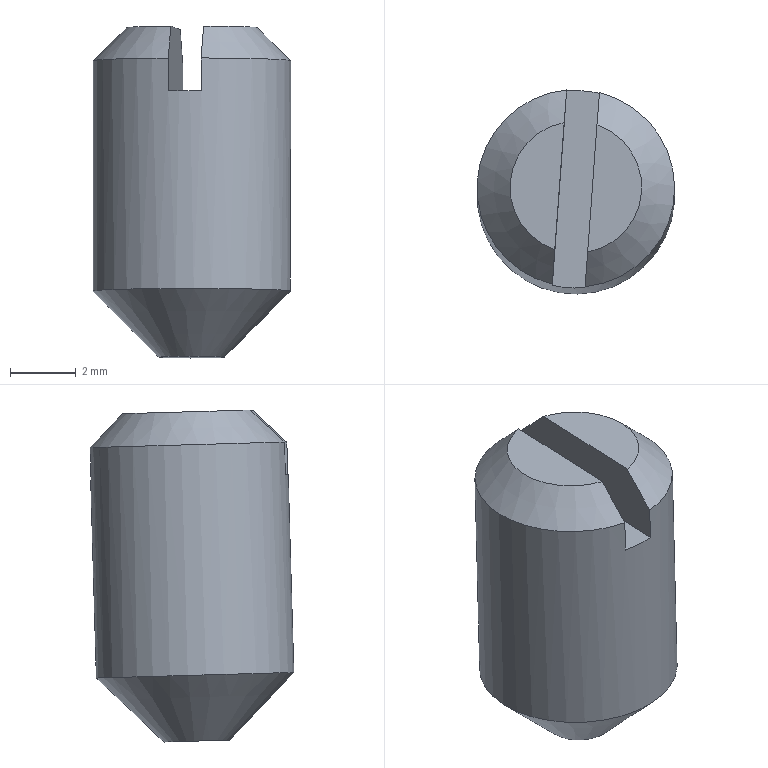Component | NX | SCREW | 1 solid | 10 faces | box 6 x 6.18 x 10.08 mm | volume 234 mm3 | plane 6 | cone 3 | cylinder 1 | commonest cylinder face diameters 6 x1
STEP:
#1=CARTESIAN_POINT('',(0.,0.,0.));
#2=DIRECTION('',(0.,0.,1.));
#3=DIRECTION('',(1.,0.,0.));
#4=AXIS2_PLACEMENT_3D('',#1,#2,#3);
#5=CARTESIAN_POINT('',(-94.356,2.396,24.438));
#6=VERTEX_POINT('',#5);
#7=CARTESIAN_POINT('',(-94.641,-1.465,24.548));
#8=VERTEX_POINT('',#7);
#9=CARTESIAN_POINT('',(-94.223,4.192,24.386));
#10=DIRECTION('',(-0.07371,-0.9969,0.02852));
#11=VECTOR('',#10,1.);
#12=LINE('',#9,#11);
#13=CARTESIAN_POINT('',(-96.992,0.6501,24.488));
#14=DIRECTION('',(0.,0.0286,0.9996));
#15=DIRECTION('',(0.9973,-0.07368,0.002108));
#16=AXIS2_PLACEMENT_3D('',#13,#14,#15);
#17=PLANE('',#16);
#18=CARTESIAN_POINT('',(2.5,3.737));
#19=DIRECTION('',(-0.,-1.));
#20=VECTOR('',#19,1.);
#21=LINE('',#18,#20);
#22=(GEOMETRIC_REPRESENTATION_CONTEXT(2)PARAMETRIC_REPRESENTATION_CONTEXT()REPRESENTATION_CONTEXT('',''));
#23=DEFINITIONAL_REPRESENTATION('',(#21),#22);
#24=PCURVE('',#17,#23);
#25=CARTESIAN_POINT('',(-94.223,4.134,22.387));
#26=DIRECTION('',(-0.9973,0.07368,-0.002108));
#27=DIRECTION('',(0.07371,0.9969,-0.02852));
#28=AXIS2_PLACEMENT_3D('',#25,#26,#27);
#29=PLANE('',#28);
#30=CARTESIAN_POINT('',(-0.,-2.));
#31=DIRECTION('',(-1.,0.));
#32=VECTOR('',#31,1.);
#33=LINE('',#30,#32);
#34=(GEOMETRIC_REPRESENTATION_CONTEXT(2)PARAMETRIC_REPRESENTATION_CONTEXT()REPRESENTATION_CONTEXT('',''));
#35=DEFINITIONAL_REPRESENTATION('',(#33),#34);
#36=PCURVE('',#29,#35);
#37=SURFACE_CURVE('',#12,(#24,#36),.PCURVE_S1.);
#38=EDGE_CURVE('',#6,#8,#37,.T.);
#39=ORIENTED_EDGE('',*,*,#38,.F.);
#40=CARTESIAN_POINT('',(-94.,0.429,24.494));
#41=DIRECTION('',(0.,0.0286,0.9996));
#42=DIRECTION('',(0.9973,-0.07368,0.002108));
#43=AXIS2_PLACEMENT_3D('',#40,#41,#42);
#44=CIRCLE('',#43,2.);
#45=CARTESIAN_POINT('',(3.,-0.));
#46=DIRECTION('',(1.,-0.));
#47=AXIS2_PLACEMENT_2D('',#45,#46);
#48=CIRCLE('',#47,2.);
#49=(GEOMETRIC_REPRESENTATION_CONTEXT(2)PARAMETRIC_REPRESENTATION_CONTEXT()REPRESENTATION_CONTEXT('',''));
#50=DEFINITIONAL_REPRESENTATION('',(#48),#49);
#51=PCURVE('',#17,#50);
#52=CARTESIAN_POINT('',(-94.,0.4004,23.494));
#53=DIRECTION('',(0.,-0.0286,-0.9996));
#54=DIRECTION('',(-0.9973,0.07368,-0.002108));
#55=AXIS2_PLACEMENT_3D('',#52,#53,#54);
#56=CONICAL_SURFACE('',#55,3.,0.7854);
#57=CARTESIAN_POINT('',(9.425,-1.));
#58=DIRECTION('',(-1.,-0.));
#59=VECTOR('',#58,1.);
#60=LINE('',#57,#59);
#61=(GEOMETRIC_REPRESENTATION_CONTEXT(2)PARAMETRIC_REPRESENTATION_CONTEXT()REPRESENTATION_CONTEXT('',''));
#62=DEFINITIONAL_REPRESENTATION('',(#60),#61);
#63=PCURVE('',#56,#62);
#64=SURFACE_CURVE('',#44,(#51,#63),.PCURVE_S1.);
#65=EDGE_CURVE('',#6,#8,#64,.T.);
#66=ORIENTED_EDGE('',*,*,#65,.T.);
#67=EDGE_LOOP('',(#39,#66));
#68=FACE_BOUND('',#67,.T.);
#69=ADVANCED_FACE('',(#68),#17,.T.);
#70=CARTESIAN_POINT('',(-93.644,-1.538,24.55));
#71=VERTEX_POINT('',#70);
#72=CARTESIAN_POINT('',(-93.359,2.323,24.44));
#73=VERTEX_POINT('',#72);
#74=CARTESIAN_POINT('',(-93.777,-3.334,24.602));
#75=DIRECTION('',(0.07371,0.9969,-0.02852));
#76=VECTOR('',#75,1.);
#77=LINE('',#74,#76);
#78=CARTESIAN_POINT('',(-96.992,0.6501,24.488));
#79=DIRECTION('',(0.,0.0286,0.9996));
#80=DIRECTION('',(0.9973,-0.07368,0.002108));
#81=AXIS2_PLACEMENT_3D('',#78,#79,#80);
#82=PLANE('',#81);
#83=CARTESIAN_POINT('',(3.5,-3.737));
#84=DIRECTION('',(0.,1.));
#85=VECTOR('',#84,1.);
#86=LINE('',#83,#85);
#87=(GEOMETRIC_REPRESENTATION_CONTEXT(2)PARAMETRIC_REPRESENTATION_CONTEXT()REPRESENTATION_CONTEXT('',''));
#88=DEFINITIONAL_REPRESENTATION('',(#86),#87);
#89=PCURVE('',#82,#88);
#90=CARTESIAN_POINT('',(-93.777,-3.391,22.602));
#91=DIRECTION('',(0.9973,-0.07368,0.002108));
#92=DIRECTION('',(-0.07371,-0.9969,0.02852));
#93=AXIS2_PLACEMENT_3D('',#90,#91,#92);
#94=PLANE('',#93);
#95=CARTESIAN_POINT('',(0.,-2.));
#96=DIRECTION('',(-1.,-0.));
#97=VECTOR('',#96,1.);
#98=LINE('',#95,#97);
#99=(GEOMETRIC_REPRESENTATION_CONTEXT(2)PARAMETRIC_REPRESENTATION_CONTEXT()REPRESENTATION_CONTEXT('',''));
#100=DEFINITIONAL_REPRESENTATION('',(#98),#99);
#101=PCURVE('',#94,#100);
#102=SURFACE_CURVE('',#77,(#89,#101),.PCURVE_S1.);
#103=EDGE_CURVE('',#71,#73,#102,.T.);
#104=ORIENTED_EDGE('',*,*,#103,.F.);
#105=CARTESIAN_POINT('',(-94.,0.429,24.494));
#106=DIRECTION('',(0.,0.0286,0.9996));
#107=DIRECTION('',(0.9973,-0.07368,0.002108));
#108=AXIS2_PLACEMENT_3D('',#105,#106,#107);
#109=CIRCLE('',#108,2.);
#110=CARTESIAN_POINT('',(3.,-0.));
#111=DIRECTION('',(1.,-0.));
#112=AXIS2_PLACEMENT_2D('',#110,#111);
#113=CIRCLE('',#112,2.);
#114=(GEOMETRIC_REPRESENTATION_CONTEXT(2)PARAMETRIC_REPRESENTATION_CONTEXT()REPRESENTATION_CONTEXT('',''));
#115=DEFINITIONAL_REPRESENTATION('',(#113),#114);
#116=PCURVE('',#82,#115);
#117=CARTESIAN_POINT('',(-94.,0.4004,23.494));
#118=DIRECTION('',(0.,-0.0286,-0.9996));
#119=DIRECTION('',(-0.9973,0.07368,-0.002108));
#120=AXIS2_PLACEMENT_3D('',#117,#118,#119);
#121=CONICAL_SURFACE('',#120,3.,0.7854);
#122=CARTESIAN_POINT('',(9.425,-1.));
#123=DIRECTION('',(-1.,0.));
#124=VECTOR('',#123,1.);
#125=LINE('',#122,#124);
#126=(GEOMETRIC_REPRESENTATION_CONTEXT(2)PARAMETRIC_REPRESENTATION_CONTEXT()REPRESENTATION_CONTEXT('',''));
#127=DEFINITIONAL_REPRESENTATION('',(#125),#126);
#128=PCURVE('',#121,#127);
#129=SURFACE_CURVE('',#109,(#116,#128),.PCURVE_S1.);
#130=EDGE_CURVE('',#71,#73,#129,.T.);
#131=ORIENTED_EDGE('',*,*,#130,.T.);
#132=EDGE_LOOP('',(#104,#131));
#133=FACE_BOUND('',#132,.T.);
#134=ADVANCED_FACE('',(#133),#82,.T.);
#135=CARTESIAN_POINT('',(-94.717,-2.512,23.578));
#136=VERTEX_POINT('',#135);
#137=CARTESIAN_POINT('',(-94.717,-2.54,22.578));
#138=VERTEX_POINT('',#137);
#139=CARTESIAN_POINT('',(-94.717,-2.769,14.581));
#140=DIRECTION('',(0.,-0.0286,-0.9996));
#141=VECTOR('',#140,1.);
#142=LINE('',#139,#141);
#143=CARTESIAN_POINT('',(-94.,0.143,14.498));
#144=DIRECTION('',(0.,-0.0286,-0.9996));
#145=DIRECTION('',(-0.9973,0.07368,-0.002108));
#146=AXIS2_PLACEMENT_3D('',#143,#144,#145);
#147=CYLINDRICAL_SURFACE('',#146,3.);
#148=CARTESIAN_POINT('',(4.88,0.));
#149=DIRECTION('',(0.,1.));
#150=VECTOR('',#149,1.);
#151=LINE('',#148,#150);
#152=(GEOMETRIC_REPRESENTATION_CONTEXT(2)PARAMETRIC_REPRESENTATION_CONTEXT()REPRESENTATION_CONTEXT('',''));
#153=DEFINITIONAL_REPRESENTATION('',(#151),#152);
#154=PCURVE('',#147,#153);
#155=CARTESIAN_POINT('',(-6.695,8.));
#156=DIRECTION('',(0.,1.));
#157=VECTOR('',#156,1.);
#158=LINE('',#155,#157);
#159=(GEOMETRIC_REPRESENTATION_CONTEXT(2)PARAMETRIC_REPRESENTATION_CONTEXT()REPRESENTATION_CONTEXT('',''));
#160=DEFINITIONAL_REPRESENTATION('',(#158),#159);
#161=PCURVE('',#29,#160);
#162=SURFACE_CURVE('',#142,(#154,#161),.PCURVE_S1.);
#163=EDGE_CURVE('',#136,#138,#162,.T.);
#164=ORIENTED_EDGE('',*,*,#163,.F.);
#165=CARTESIAN_POINT('',(-96.992,0.6215,23.488));
#166=VERTEX_POINT('',#165);
#167=CARTESIAN_POINT('',(-94.,0.4004,23.494));
#168=DIRECTION('',(0.,-0.0286,-0.9996));
#169=DIRECTION('',(0.9973,-0.07368,0.002108));
#170=AXIS2_PLACEMENT_3D('',#167,#168,#169);
#171=CIRCLE('',#170,3.);
#172=CARTESIAN_POINT('',(3.142,-9.));
#173=DIRECTION('',(1.,0.));
#174=VECTOR('',#173,1.);
#175=LINE('',#172,#174);
#176=(GEOMETRIC_REPRESENTATION_CONTEXT(2)PARAMETRIC_REPRESENTATION_CONTEXT()REPRESENTATION_CONTEXT('',''));
#177=DEFINITIONAL_REPRESENTATION('',(#175),#176);
#178=PCURVE('',#147,#177);
#179=CARTESIAN_POINT('',(3.142,-0.));
#180=DIRECTION('',(1.,0.));
#181=VECTOR('',#180,1.);
#182=LINE('',#179,#181);
#183=(GEOMETRIC_REPRESENTATION_CONTEXT(2)PARAMETRIC_REPRESENTATION_CONTEXT()REPRESENTATION_CONTEXT('',''));
#184=DEFINITIONAL_REPRESENTATION('',(#182),#183);
#185=PCURVE('',#56,#184);
#186=SURFACE_CURVE('',#171,(#178,#185),.PCURVE_S1.);
#187=EDGE_CURVE('',#136,#166,#186,.T.);
#188=ORIENTED_EDGE('',*,*,#187,.T.);
#189=CARTESIAN_POINT('',(-96.992,0.4212,16.491));
#190=VERTEX_POINT('',#189);
#191=CARTESIAN_POINT('',(-96.992,0.6215,23.488));
#192=CARTESIAN_POINT('',(-96.992,0.4212,16.491));
#193=B_SPLINE_CURVE_WITH_KNOTS('',1,(#191,#192),.UNSPECIFIED.,.F.,.F.,(2,2),(-9.,-2.),.PIECEWISE_BEZIER_KNOTS.);
#194=CARTESIAN_POINT('',(6.283,0.));
#195=DIRECTION('',(0.,1.));
#196=VECTOR('',#195,1.);
#197=LINE('',#194,#196);
#198=(GEOMETRIC_REPRESENTATION_CONTEXT(2)PARAMETRIC_REPRESENTATION_CONTEXT()REPRESENTATION_CONTEXT('',''));
#199=DEFINITIONAL_REPRESENTATION('',(#197),#198);
#200=PCURVE('',#147,#199);
#201=CARTESIAN_POINT('',(0.,0.));
#202=DIRECTION('',(0.,1.));
#203=VECTOR('',#202,1.);
#204=LINE('',#201,#203);
#205=(GEOMETRIC_REPRESENTATION_CONTEXT(2)PARAMETRIC_REPRESENTATION_CONTEXT()REPRESENTATION_CONTEXT('',''));
#206=DEFINITIONAL_REPRESENTATION('',(#204),#205);
#207=PCURVE('',#147,#206);
#208=SEAM_CURVE('',#193,(#200,#207),.PCURVE_S1.);
#209=EDGE_CURVE('',#166,#190,#208,.T.);
#210=ORIENTED_EDGE('',*,*,#209,.T.);
#211=CARTESIAN_POINT('',(-94.,0.2002,16.497));
#212=DIRECTION('',(0.,-0.0286,-0.9996));
#213=DIRECTION('',(-0.9973,0.07368,-0.002108));
#214=AXIS2_PLACEMENT_3D('',#211,#212,#213);
#215=CIRCLE('',#214,3.);
#216=CARTESIAN_POINT('',(0.,-2.));
#217=DIRECTION('',(1.,0.));
#218=VECTOR('',#217,1.);
#219=LINE('',#216,#218);
#220=(GEOMETRIC_REPRESENTATION_CONTEXT(2)PARAMETRIC_REPRESENTATION_CONTEXT()REPRESENTATION_CONTEXT('',''));
#221=DEFINITIONAL_REPRESENTATION('',(#219),#220);
#222=PCURVE('',#147,#221);
#223=CARTESIAN_POINT('',(-94.,0.143,14.498));
#224=DIRECTION('',(0.,0.0286,0.9996));
#225=DIRECTION('',(0.9973,-0.07368,0.002108));
#226=AXIS2_PLACEMENT_3D('',#223,#224,#225);
#227=CONICAL_SURFACE('',#226,1.,0.7854);
#228=CARTESIAN_POINT('',(9.425,2.));
#229=DIRECTION('',(-1.,0.));
#230=VECTOR('',#229,1.);
#231=LINE('',#228,#230);
#232=(GEOMETRIC_REPRESENTATION_CONTEXT(2)PARAMETRIC_REPRESENTATION_CONTEXT()REPRESENTATION_CONTEXT('',''));
#233=DEFINITIONAL_REPRESENTATION('',(#231),#232);
#234=PCURVE('',#227,#233);
#235=SURFACE_CURVE('',#215,(#222,#234),.PCURVE_S1.);
#236=EDGE_CURVE('',#190,#190,#235,.T.);
#237=ORIENTED_EDGE('',*,*,#236,.F.);
#238=ORIENTED_EDGE('',*,*,#209,.F.);
#239=CARTESIAN_POINT('',(-94.281,3.386,23.409));
#240=VERTEX_POINT('',#239);
#241=CARTESIAN_POINT('',(-94.,0.4004,23.494));
#242=DIRECTION('',(0.,-0.0286,-0.9996));
#243=DIRECTION('',(0.9973,-0.07368,0.002108));
#244=AXIS2_PLACEMENT_3D('',#241,#242,#243);
#245=CIRCLE('',#244,3.);
#246=CARTESIAN_POINT('',(-3.142,-9.));
#247=DIRECTION('',(1.,0.));
#248=VECTOR('',#247,1.);
#249=LINE('',#246,#248);
#250=(GEOMETRIC_REPRESENTATION_CONTEXT(2)PARAMETRIC_REPRESENTATION_CONTEXT()REPRESENTATION_CONTEXT('',''));
#251=DEFINITIONAL_REPRESENTATION('',(#249),#250);
#252=PCURVE('',#147,#251);
#253=CARTESIAN_POINT('',(3.142,0.));
#254=DIRECTION('',(1.,-0.));
#255=VECTOR('',#254,1.);
#256=LINE('',#253,#255);
#257=(GEOMETRIC_REPRESENTATION_CONTEXT(2)PARAMETRIC_REPRESENTATION_CONTEXT()REPRESENTATION_CONTEXT('',''));
#258=DEFINITIONAL_REPRESENTATION('',(#256),#257);
#259=PCURVE('',#56,#258);
#260=SURFACE_CURVE('',#245,(#252,#259),.PCURVE_S1.);
#261=EDGE_CURVE('',#166,#240,#260,.T.);
#262=ORIENTED_EDGE('',*,*,#261,.T.);
#263=CARTESIAN_POINT('',(-94.281,3.357,22.409));
#264=VERTEX_POINT('',#263);
#265=CARTESIAN_POINT('',(-94.281,3.129,14.413));
#266=DIRECTION('',(0.,0.0286,0.9996));
#267=VECTOR('',#266,1.);
#268=LINE('',#265,#267);
#269=CARTESIAN_POINT('',(1.403,0.));
#270=DIRECTION('',(0.,-1.));
#271=VECTOR('',#270,1.);
#272=LINE('',#269,#271);
#273=(GEOMETRIC_REPRESENTATION_CONTEXT(2)PARAMETRIC_REPRESENTATION_CONTEXT()REPRESENTATION_CONTEXT('',''));
#274=DEFINITIONAL_REPRESENTATION('',(#272),#273);
#275=PCURVE('',#147,#274);
#276=CARTESIAN_POINT('',(-0.7794,8.));
#277=DIRECTION('',(-0.,-1.));
#278=VECTOR('',#277,1.);
#279=LINE('',#276,#278);
#280=(GEOMETRIC_REPRESENTATION_CONTEXT(2)PARAMETRIC_REPRESENTATION_CONTEXT()REPRESENTATION_CONTEXT('',''));
#281=DEFINITIONAL_REPRESENTATION('',(#279),#280);
#282=PCURVE('',#29,#281);
#283=SURFACE_CURVE('',#268,(#275,#282),.PCURVE_S1.);
#284=EDGE_CURVE('',#264,#240,#283,.T.);
#285=ORIENTED_EDGE('',*,*,#284,.F.);
#286=CARTESIAN_POINT('',(-93.283,3.284,22.411));
#287=VERTEX_POINT('',#286);
#288=CARTESIAN_POINT('',(-94.,0.3718,22.495));
#289=DIRECTION('',(0.,-0.0286,-0.9996));
#290=DIRECTION('',(0.9973,-0.07368,0.002108));
#291=AXIS2_PLACEMENT_3D('',#288,#289,#290);
#292=CIRCLE('',#291,3.);
#293=CARTESIAN_POINT('',(-3.142,-8.));
#294=DIRECTION('',(1.,0.));
#295=VECTOR('',#294,1.);
#296=LINE('',#293,#295);
#297=(GEOMETRIC_REPRESENTATION_CONTEXT(2)PARAMETRIC_REPRESENTATION_CONTEXT()REPRESENTATION_CONTEXT('',''));
#298=DEFINITIONAL_REPRESENTATION('',(#296),#297);
#299=PCURVE('',#147,#298);
#300=CARTESIAN_POINT('',(-94.,0.3718,22.495));
#301=DIRECTION('',(0.,0.0286,0.9996));
#302=DIRECTION('',(0.9973,-0.07368,0.002108));
#303=AXIS2_PLACEMENT_3D('',#300,#301,#302);
#304=PLANE('',#303);
#305=CARTESIAN_POINT('',(3.,-0.));
#306=CARTESIAN_POINT('',(3.,-5.196));
#307=CARTESIAN_POINT('',(-1.5,-2.598));
#308=CARTESIAN_POINT('',(-6.,0.));
#309=CARTESIAN_POINT('',(-1.5,2.598));
#310=CARTESIAN_POINT('',(3.,5.196));
#311=CARTESIAN_POINT('',(3.,-0.));
#312=(BOUNDED_CURVE()B_SPLINE_CURVE(2,(#305,#306,#307,#308,#309,#310,#311),.UNSPECIFIED.,.T.,.F.)B_SPLINE_CURVE_WITH_KNOTS((1,2,2,2,2,1),(-2.094,0.,2.094,4.189,6.283,8.378),.UNSPECIFIED.)CURVE()GEOMETRIC_REPRESENTATION_ITEM()RATIONAL_B_SPLINE_CURVE((1.,0.5,1.,0.5,1.,0.5,1.))REPRESENTATION_ITEM(''));
#313=(GEOMETRIC_REPRESENTATION_CONTEXT(2)PARAMETRIC_REPRESENTATION_CONTEXT()REPRESENTATION_CONTEXT('',''));
#314=DEFINITIONAL_REPRESENTATION('',(#312),#313);
#315=PCURVE('',#304,#314);
#316=SURFACE_CURVE('',#292,(#299,#315),.PCURVE_S1.);
#317=EDGE_CURVE('',#264,#287,#316,.T.);
#318=ORIENTED_EDGE('',*,*,#317,.T.);
#319=CARTESIAN_POINT('',(-93.283,3.312,23.411));
#320=VERTEX_POINT('',#319);
#321=CARTESIAN_POINT('',(-93.283,3.055,14.415));
#322=DIRECTION('',(0.,-0.0286,-0.9996));
#323=VECTOR('',#322,1.);
#324=LINE('',#321,#323);
#325=CARTESIAN_POINT('',(1.738,0.));
#326=DIRECTION('',(0.,1.));
#327=VECTOR('',#326,1.);
#328=LINE('',#325,#327);
#329=(GEOMETRIC_REPRESENTATION_CONTEXT(2)PARAMETRIC_REPRESENTATION_CONTEXT()REPRESENTATION_CONTEXT('',''));
#330=DEFINITIONAL_REPRESENTATION('',(#328),#329);
#331=PCURVE('',#147,#330);
#332=CARTESIAN_POINT('',(-6.695,8.));
#333=DIRECTION('',(-0.,1.));
#334=VECTOR('',#333,1.);
#335=LINE('',#332,#334);
#336=(GEOMETRIC_REPRESENTATION_CONTEXT(2)PARAMETRIC_REPRESENTATION_CONTEXT()REPRESENTATION_CONTEXT('',''));
#337=DEFINITIONAL_REPRESENTATION('',(#335),#336);
#338=PCURVE('',#94,#337);
#339=SURFACE_CURVE('',#324,(#331,#338),.PCURVE_S1.);
#340=EDGE_CURVE('',#320,#287,#339,.T.);
#341=ORIENTED_EDGE('',*,*,#340,.F.);
#342=CARTESIAN_POINT('',(-93.719,-2.585,23.58));
#343=VERTEX_POINT('',#342);
#344=CARTESIAN_POINT('',(-94.,0.4004,23.494));
#345=DIRECTION('',(0.,-0.0286,-0.9996));
#346=DIRECTION('',(0.9973,-0.07368,0.002108));
#347=AXIS2_PLACEMENT_3D('',#344,#345,#346);
#348=CIRCLE('',#347,3.);
#349=CARTESIAN_POINT('',(-3.142,-9.));
#350=DIRECTION('',(1.,0.));
#351=VECTOR('',#350,1.);
#352=LINE('',#349,#351);
#353=(GEOMETRIC_REPRESENTATION_CONTEXT(2)PARAMETRIC_REPRESENTATION_CONTEXT()REPRESENTATION_CONTEXT('',''));
#354=DEFINITIONAL_REPRESENTATION('',(#352),#353);
#355=PCURVE('',#147,#354);
#356=CARTESIAN_POINT('',(-3.142,-0.));
#357=DIRECTION('',(1.,0.));
#358=VECTOR('',#357,1.);
#359=LINE('',#356,#358);
#360=(GEOMETRIC_REPRESENTATION_CONTEXT(2)PARAMETRIC_REPRESENTATION_CONTEXT()REPRESENTATION_CONTEXT('',''));
#361=DEFINITIONAL_REPRESENTATION('',(#359),#360);
#362=PCURVE('',#121,#361);
#363=SURFACE_CURVE('',#348,(#355,#362),.PCURVE_S1.);
#364=EDGE_CURVE('',#320,#343,#363,.T.);
#365=ORIENTED_EDGE('',*,*,#364,.T.);
#366=CARTESIAN_POINT('',(-93.719,-2.614,22.58));
#367=VERTEX_POINT('',#366);
#368=CARTESIAN_POINT('',(-93.719,-2.843,14.583));
#369=DIRECTION('',(0.,0.0286,0.9996));
#370=VECTOR('',#369,1.);
#371=LINE('',#368,#370);
#372=CARTESIAN_POINT('',(4.545,0.));
#373=DIRECTION('',(-0.,-1.));
#374=VECTOR('',#373,1.);
#375=LINE('',#372,#374);
#376=(GEOMETRIC_REPRESENTATION_CONTEXT(2)PARAMETRIC_REPRESENTATION_CONTEXT()REPRESENTATION_CONTEXT('',''));
#377=DEFINITIONAL_REPRESENTATION('',(#375),#376);
#378=PCURVE('',#147,#377);
#379=CARTESIAN_POINT('',(-0.7794,8.));
#380=DIRECTION('',(0.,-1.));
#381=VECTOR('',#380,1.);
#382=LINE('',#379,#381);
#383=(GEOMETRIC_REPRESENTATION_CONTEXT(2)PARAMETRIC_REPRESENTATION_CONTEXT()REPRESENTATION_CONTEXT('',''));
#384=DEFINITIONAL_REPRESENTATION('',(#382),#383);
#385=PCURVE('',#94,#384);
#386=SURFACE_CURVE('',#371,(#378,#385),.PCURVE_S1.);
#387=EDGE_CURVE('',#367,#343,#386,.T.);
#388=ORIENTED_EDGE('',*,*,#387,.F.);
#389=CARTESIAN_POINT('',(-94.,0.3718,22.495));
#390=DIRECTION('',(0.,-0.0286,-0.9996));
#391=DIRECTION('',(0.9973,-0.07368,0.002108));
#392=AXIS2_PLACEMENT_3D('',#389,#390,#391);
#393=CIRCLE('',#392,3.);
#394=CARTESIAN_POINT('',(3.142,-8.));
#395=DIRECTION('',(1.,0.));
#396=VECTOR('',#395,1.);
#397=LINE('',#394,#396);
#398=(GEOMETRIC_REPRESENTATION_CONTEXT(2)PARAMETRIC_REPRESENTATION_CONTEXT()REPRESENTATION_CONTEXT('',''));
#399=DEFINITIONAL_REPRESENTATION('',(#397),#398);
#400=PCURVE('',#147,#399);
#401=CARTESIAN_POINT('',(3.,-0.));
#402=CARTESIAN_POINT('',(3.,-5.196));
#403=CARTESIAN_POINT('',(-1.5,-2.598));
#404=CARTESIAN_POINT('',(-6.,0.));
#405=CARTESIAN_POINT('',(-1.5,2.598));
#406=CARTESIAN_POINT('',(3.,5.196));
#407=CARTESIAN_POINT('',(3.,-0.));
#408=(BOUNDED_CURVE()B_SPLINE_CURVE(2,(#401,#402,#403,#404,#405,#406,#407),.UNSPECIFIED.,.T.,.F.)B_SPLINE_CURVE_WITH_KNOTS((1,2,2,2,2,1),(-2.094,0.,2.094,4.189,6.283,8.378),.UNSPECIFIED.)CURVE()GEOMETRIC_REPRESENTATION_ITEM()RATIONAL_B_SPLINE_CURVE((1.,0.5,1.,0.5,1.,0.5,1.))REPRESENTATION_ITEM(''));
#409=(GEOMETRIC_REPRESENTATION_CONTEXT(2)PARAMETRIC_REPRESENTATION_CONTEXT()REPRESENTATION_CONTEXT('',''));
#410=DEFINITIONAL_REPRESENTATION('',(#408),#409);
#411=PCURVE('',#304,#410);
#412=SURFACE_CURVE('',#393,(#400,#411),.PCURVE_S1.);
#413=EDGE_CURVE('',#367,#138,#412,.T.);
#414=ORIENTED_EDGE('',*,*,#413,.T.);
#415=EDGE_LOOP('',(#164,#188,#210,#237,#238,#262,#285,#318,#341,#365,#388,#414));
#416=FACE_BOUND('',#415,.T.);
#417=ADVANCED_FACE('',(#416),#147,.T.);
#418=ORIENTED_EDGE('',*,*,#236,.T.);
#419=CARTESIAN_POINT('',(-94.997,0.2167,14.496));
#420=VERTEX_POINT('',#419);
#421=CARTESIAN_POINT('',(-94.997,0.2167,14.496));
#422=CARTESIAN_POINT('',(-96.992,0.4212,16.491));
#423=B_SPLINE_CURVE_WITH_KNOTS('',1,(#421,#422),.UNSPECIFIED.,.F.,.F.,(2,2),(0.,2.828),.PIECEWISE_BEZIER_KNOTS.);
#424=CARTESIAN_POINT('',(3.142,0.));
#425=DIRECTION('',(0.,1.));
#426=VECTOR('',#425,1.);
#427=LINE('',#424,#426);
#428=(GEOMETRIC_REPRESENTATION_CONTEXT(2)PARAMETRIC_REPRESENTATION_CONTEXT()REPRESENTATION_CONTEXT('',''));
#429=DEFINITIONAL_REPRESENTATION('',(#427),#428);
#430=PCURVE('',#227,#429);
#431=CARTESIAN_POINT('',(9.425,0.));
#432=DIRECTION('',(0.,1.));
#433=VECTOR('',#432,1.);
#434=LINE('',#431,#433);
#435=(GEOMETRIC_REPRESENTATION_CONTEXT(2)PARAMETRIC_REPRESENTATION_CONTEXT()REPRESENTATION_CONTEXT('',''));
#436=DEFINITIONAL_REPRESENTATION('',(#434),#435);
#437=PCURVE('',#227,#436);
#438=SEAM_CURVE('',#423,(#430,#437),.PCURVE_S1.);
#439=EDGE_CURVE('',#420,#190,#438,.T.);
#440=ORIENTED_EDGE('',*,*,#439,.F.);
#441=CARTESIAN_POINT('',(-94.,0.143,14.498));
#442=DIRECTION('',(0.,-0.0286,-0.9996));
#443=DIRECTION('',(-0.9973,0.07368,-0.002108));
#444=AXIS2_PLACEMENT_3D('',#441,#442,#443);
#445=CIRCLE('',#444,1.);
#446=CARTESIAN_POINT('',(9.425,0.));
#447=DIRECTION('',(-1.,0.));
#448=VECTOR('',#447,1.);
#449=LINE('',#446,#448);
#450=(GEOMETRIC_REPRESENTATION_CONTEXT(2)PARAMETRIC_REPRESENTATION_CONTEXT()REPRESENTATION_CONTEXT('',''));
#451=DEFINITIONAL_REPRESENTATION('',(#449),#450);
#452=PCURVE('',#227,#451);
#453=CARTESIAN_POINT('',(-94.,0.143,14.498));
#454=DIRECTION('',(0.,-0.0286,-0.9996));
#455=DIRECTION('',(-0.9973,0.07368,-0.002108));
#456=AXIS2_PLACEMENT_3D('',#453,#454,#455);
#457=PLANE('',#456);
#458=CARTESIAN_POINT('',(0.,0.));
#459=DIRECTION('',(1.,0.));
#460=AXIS2_PLACEMENT_2D('',#458,#459);
#461=CIRCLE('',#460,1.);
#462=(GEOMETRIC_REPRESENTATION_CONTEXT(2)PARAMETRIC_REPRESENTATION_CONTEXT()REPRESENTATION_CONTEXT('',''));
#463=DEFINITIONAL_REPRESENTATION('',(#461),#462);
#464=PCURVE('',#457,#463);
#465=SURFACE_CURVE('',#445,(#452,#464),.PCURVE_S1.);
#466=EDGE_CURVE('',#420,#420,#465,.T.);
#467=ORIENTED_EDGE('',*,*,#466,.F.);
#468=ORIENTED_EDGE('',*,*,#439,.T.);
#469=EDGE_LOOP('',(#418,#440,#467,#468));
#470=FACE_BOUND('',#469,.T.);
#471=ADVANCED_FACE('',(#470),#227,.T.);
#472=ORIENTED_EDGE('',*,*,#466,.T.);
#473=EDGE_LOOP('',(#472));
#474=FACE_BOUND('',#473,.T.);
#475=ADVANCED_FACE('',(#474),#457,.T.);
#476=ORIENTED_EDGE('',*,*,#284,.T.);
#477=CARTESIAN_POINT('',(-94.281,3.386,23.409));
#478=CARTESIAN_POINT('',(-94.306,3.057,23.753));
#479=CARTESIAN_POINT('',(-94.331,2.728,24.096));
#480=CARTESIAN_POINT('',(-94.356,2.396,24.438));
#481=B_SPLINE_CURVE_WITH_KNOTS('',3,(#477,#478,#479,#480),.UNSPECIFIED.,.F.,.F.,(4,4),(0.,1.),.PIECEWISE_BEZIER_KNOTS.);
#482=CARTESIAN_POINT('',(-0.7794,-1.));
#483=CARTESIAN_POINT('',(-1.119,-1.335));
#484=CARTESIAN_POINT('',(-1.459,-1.669));
#485=CARTESIAN_POINT('',(-1.801,-2.));
#486=B_SPLINE_CURVE_WITH_KNOTS('',3,(#482,#483,#484,#485),.UNSPECIFIED.,.F.,.F.,(4,4),(0.,1.),.PIECEWISE_BEZIER_KNOTS.);
#487=(GEOMETRIC_REPRESENTATION_CONTEXT(2)PARAMETRIC_REPRESENTATION_CONTEXT()REPRESENTATION_CONTEXT('',''));
#488=DEFINITIONAL_REPRESENTATION('',(#486),#487);
#489=PCURVE('',#29,#488);
#490=CARTESIAN_POINT('',(7.687,-0.));
#491=CARTESIAN_POINT('',(7.601,-1.));
#492=B_SPLINE_CURVE_WITH_KNOTS('',1,(#490,#491),.UNSPECIFIED.,.F.,.F.,(2,2),(0.,1.),.PIECEWISE_BEZIER_KNOTS.);
#493=(GEOMETRIC_REPRESENTATION_CONTEXT(2)PARAMETRIC_REPRESENTATION_CONTEXT()REPRESENTATION_CONTEXT('',''));
#494=DEFINITIONAL_REPRESENTATION('',(#492),#493);
#495=PCURVE('',#56,#494);
#496=SURFACE_CURVE('',#481,(#489,#495),.PCURVE_S1.);
#497=EDGE_CURVE('',#240,#6,#496,.T.);
#498=ORIENTED_EDGE('',*,*,#497,.T.);
#499=ORIENTED_EDGE('',*,*,#38,.T.);
#500=CARTESIAN_POINT('',(-94.641,-1.465,24.548));
#501=CARTESIAN_POINT('',(-94.667,-1.815,24.226));
#502=CARTESIAN_POINT('',(-94.692,-2.164,23.902));
#503=CARTESIAN_POINT('',(-94.717,-2.512,23.578));
#504=B_SPLINE_CURVE_WITH_KNOTS('',3,(#500,#501,#502,#503),.UNSPECIFIED.,.F.,.F.,(4,4),(0.,1.),.PIECEWISE_BEZIER_KNOTS.);
#505=CARTESIAN_POINT('',(-5.674,-2.));
#506=CARTESIAN_POINT('',(-6.016,-1.669));
#507=CARTESIAN_POINT('',(-6.356,-1.335));
#508=CARTESIAN_POINT('',(-6.695,-1.));
#509=B_SPLINE_CURVE_WITH_KNOTS('',3,(#505,#506,#507,#508),.UNSPECIFIED.,.F.,.F.,(4,4),(0.,1.),.PIECEWISE_BEZIER_KNOTS.);
#510=(GEOMETRIC_REPRESENTATION_CONTEXT(2)PARAMETRIC_REPRESENTATION_CONTEXT()REPRESENTATION_CONTEXT('',''));
#511=DEFINITIONAL_REPRESENTATION('',(#509),#510);
#512=PCURVE('',#29,#511);
#513=CARTESIAN_POINT('',(4.965,-1.));
#514=CARTESIAN_POINT('',(4.88,0.));
#515=B_SPLINE_CURVE_WITH_KNOTS('',1,(#513,#514),.UNSPECIFIED.,.F.,.F.,(2,2),(0.,1.),.PIECEWISE_BEZIER_KNOTS.);
#516=(GEOMETRIC_REPRESENTATION_CONTEXT(2)PARAMETRIC_REPRESENTATION_CONTEXT()REPRESENTATION_CONTEXT('',''));
#517=DEFINITIONAL_REPRESENTATION('',(#515),#516);
#518=PCURVE('',#56,#517);
#519=SURFACE_CURVE('',#504,(#512,#518),.PCURVE_S1.);
#520=EDGE_CURVE('',#8,#136,#519,.T.);
#521=ORIENTED_EDGE('',*,*,#520,.T.);
#522=ORIENTED_EDGE('',*,*,#163,.T.);
#523=CARTESIAN_POINT('',(-94.223,4.134,22.387));
#524=DIRECTION('',(0.07371,0.9969,-0.02852));
#525=VECTOR('',#524,1.);
#526=LINE('',#523,#525);
#527=CARTESIAN_POINT('',(0.,0.));
#528=DIRECTION('',(1.,-0.));
#529=VECTOR('',#528,1.);
#530=LINE('',#527,#529);
#531=(GEOMETRIC_REPRESENTATION_CONTEXT(2)PARAMETRIC_REPRESENTATION_CONTEXT()REPRESENTATION_CONTEXT('',''));
#532=DEFINITIONAL_REPRESENTATION('',(#530),#531);
#533=PCURVE('',#29,#532);
#534=CARTESIAN_POINT('',(-0.5,3.737));
#535=DIRECTION('',(0.,1.));
#536=VECTOR('',#535,1.);
#537=LINE('',#534,#536);
#538=(GEOMETRIC_REPRESENTATION_CONTEXT(2)PARAMETRIC_REPRESENTATION_CONTEXT()REPRESENTATION_CONTEXT('',''));
#539=DEFINITIONAL_REPRESENTATION('',(#537),#538);
#540=PCURVE('',#304,#539);
#541=SURFACE_CURVE('',#526,(#533,#540),.PCURVE_S1.);
#542=EDGE_CURVE('',#138,#264,#541,.T.);
#543=ORIENTED_EDGE('',*,*,#542,.T.);
#544=EDGE_LOOP('',(#476,#498,#499,#521,#522,#543));
#545=FACE_BOUND('',#544,.T.);
#546=ADVANCED_FACE('',(#545),#29,.F.);
#547=ORIENTED_EDGE('',*,*,#387,.T.);
#548=CARTESIAN_POINT('',(-93.719,-2.585,23.58));
#549=CARTESIAN_POINT('',(-93.694,-2.237,23.904));
#550=CARTESIAN_POINT('',(-93.669,-1.889,24.229));
#551=CARTESIAN_POINT('',(-93.644,-1.538,24.55));
#552=B_SPLINE_CURVE_WITH_KNOTS('',3,(#548,#549,#550,#551),.UNSPECIFIED.,.F.,.F.,(4,4),(0.,1.),.PIECEWISE_BEZIER_KNOTS.);
#553=CARTESIAN_POINT('',(-0.7794,-1.));
#554=CARTESIAN_POINT('',(-1.119,-1.335));
#555=CARTESIAN_POINT('',(-1.459,-1.669));
#556=CARTESIAN_POINT('',(-1.801,-2.));
#557=B_SPLINE_CURVE_WITH_KNOTS('',3,(#553,#554,#555,#556),.UNSPECIFIED.,.F.,.F.,(4,4),(0.,1.),.PIECEWISE_BEZIER_KNOTS.);
#558=(GEOMETRIC_REPRESENTATION_CONTEXT(2)PARAMETRIC_REPRESENTATION_CONTEXT()REPRESENTATION_CONTEXT('',''));
#559=DEFINITIONAL_REPRESENTATION('',(#557),#558);
#560=PCURVE('',#94,#559);
#561=CARTESIAN_POINT('',(4.545,0.));
#562=CARTESIAN_POINT('',(4.46,-1.));
#563=B_SPLINE_CURVE_WITH_KNOTS('',1,(#561,#562),.UNSPECIFIED.,.F.,.F.,(2,2),(0.,1.),.PIECEWISE_BEZIER_KNOTS.);
#564=(GEOMETRIC_REPRESENTATION_CONTEXT(2)PARAMETRIC_REPRESENTATION_CONTEXT()REPRESENTATION_CONTEXT('',''));
#565=DEFINITIONAL_REPRESENTATION('',(#563),#564);
#566=PCURVE('',#121,#565);
#567=SURFACE_CURVE('',#552,(#560,#566),.PCURVE_S1.);
#568=EDGE_CURVE('',#343,#71,#567,.T.);
#569=ORIENTED_EDGE('',*,*,#568,.T.);
#570=ORIENTED_EDGE('',*,*,#103,.T.);
#571=CARTESIAN_POINT('',(-93.359,2.323,24.44));
#572=CARTESIAN_POINT('',(-93.333,2.654,24.099));
#573=CARTESIAN_POINT('',(-93.308,2.984,23.755));
#574=CARTESIAN_POINT('',(-93.283,3.312,23.411));
#575=B_SPLINE_CURVE_WITH_KNOTS('',3,(#571,#572,#573,#574),.UNSPECIFIED.,.F.,.F.,(4,4),(0.,1.),.PIECEWISE_BEZIER_KNOTS.);
#576=CARTESIAN_POINT('',(-5.674,-2.));
#577=CARTESIAN_POINT('',(-6.016,-1.669));
#578=CARTESIAN_POINT('',(-6.356,-1.335));
#579=CARTESIAN_POINT('',(-6.695,-1.));
#580=B_SPLINE_CURVE_WITH_KNOTS('',3,(#576,#577,#578,#579),.UNSPECIFIED.,.F.,.F.,(4,4),(0.,1.),.PIECEWISE_BEZIER_KNOTS.);
#581=(GEOMETRIC_REPRESENTATION_CONTEXT(2)PARAMETRIC_REPRESENTATION_CONTEXT()REPRESENTATION_CONTEXT('',''));
#582=DEFINITIONAL_REPRESENTATION('',(#580),#581);
#583=PCURVE('',#94,#582);
#584=CARTESIAN_POINT('',(1.823,-1.));
#585=CARTESIAN_POINT('',(1.738,0.));
#586=B_SPLINE_CURVE_WITH_KNOTS('',1,(#584,#585),.UNSPECIFIED.,.F.,.F.,(2,2),(0.,1.),.PIECEWISE_BEZIER_KNOTS.);
#587=(GEOMETRIC_REPRESENTATION_CONTEXT(2)PARAMETRIC_REPRESENTATION_CONTEXT()REPRESENTATION_CONTEXT('',''));
#588=DEFINITIONAL_REPRESENTATION('',(#586),#587);
#589=PCURVE('',#121,#588);
#590=SURFACE_CURVE('',#575,(#583,#589),.PCURVE_S1.);
#591=EDGE_CURVE('',#73,#320,#590,.T.);
#592=ORIENTED_EDGE('',*,*,#591,.T.);
#593=ORIENTED_EDGE('',*,*,#340,.T.);
#594=CARTESIAN_POINT('',(-93.777,-3.391,22.602));
#595=DIRECTION('',(-0.07371,-0.9969,0.02852));
#596=VECTOR('',#595,1.);
#597=LINE('',#594,#596);
#598=CARTESIAN_POINT('',(0.,0.));
#599=DIRECTION('',(1.,0.));
#600=VECTOR('',#599,1.);
#601=LINE('',#598,#600);
#602=(GEOMETRIC_REPRESENTATION_CONTEXT(2)PARAMETRIC_REPRESENTATION_CONTEXT()REPRESENTATION_CONTEXT('',''));
#603=DEFINITIONAL_REPRESENTATION('',(#601),#602);
#604=PCURVE('',#94,#603);
#605=CARTESIAN_POINT('',(0.5,-3.737));
#606=DIRECTION('',(-0.,-1.));
#607=VECTOR('',#606,1.);
#608=LINE('',#605,#607);
#609=(GEOMETRIC_REPRESENTATION_CONTEXT(2)PARAMETRIC_REPRESENTATION_CONTEXT()REPRESENTATION_CONTEXT('',''));
#610=DEFINITIONAL_REPRESENTATION('',(#608),#609);
#611=PCURVE('',#304,#610);
#612=SURFACE_CURVE('',#597,(#604,#611),.PCURVE_S1.);
#613=EDGE_CURVE('',#287,#367,#612,.T.);
#614=ORIENTED_EDGE('',*,*,#613,.T.);
#615=EDGE_LOOP('',(#547,#569,#570,#592,#593,#614));
#616=FACE_BOUND('',#615,.T.);
#617=ADVANCED_FACE('',(#616),#94,.F.);
#618=ORIENTED_EDGE('',*,*,#613,.F.);
#619=ORIENTED_EDGE('',*,*,#317,.F.);
#620=ORIENTED_EDGE('',*,*,#542,.F.);
#621=ORIENTED_EDGE('',*,*,#413,.F.);
#622=EDGE_LOOP('',(#618,#619,#620,#621));
#623=FACE_BOUND('',#622,.T.);
#624=ADVANCED_FACE('',(#623),#304,.T.);
#625=ORIENTED_EDGE('',*,*,#520,.F.);
#626=ORIENTED_EDGE('',*,*,#65,.F.);
#627=ORIENTED_EDGE('',*,*,#497,.F.);
#628=ORIENTED_EDGE('',*,*,#261,.F.);
#629=ORIENTED_EDGE('',*,*,#187,.F.);
#630=EDGE_LOOP('',(#625,#626,#627,#628,#629));
#631=FACE_BOUND('',#630,.T.);
#632=ADVANCED_FACE('',(#631),#56,.T.);
#633=ORIENTED_EDGE('',*,*,#591,.F.);
#634=ORIENTED_EDGE('',*,*,#130,.F.);
#635=ORIENTED_EDGE('',*,*,#568,.F.);
#636=ORIENTED_EDGE('',*,*,#364,.F.);
#637=EDGE_LOOP('',(#633,#634,#635,#636));
#638=FACE_BOUND('',#637,.T.);
#639=ADVANCED_FACE('',(#638),#121,.T.);
#640=CLOSED_SHELL('',(#69,#134,#417,#471,#475,#546,#617,#624,#632,#639));
#641=MANIFOLD_SOLID_BREP('',#640);
#642=(LENGTH_UNIT()NAMED_UNIT(*)SI_UNIT(.MILLI.,.METRE.));
#643=UNCERTAINTY_MEASURE_WITH_UNIT(LENGTH_MEASURE(0.01),#642,'','');
#644=(NAMED_UNIT(*)PLANE_ANGLE_UNIT()SI_UNIT($,.RADIAN.));
#645=(NAMED_UNIT(*)SI_UNIT($,.STERADIAN.)SOLID_ANGLE_UNIT());
#646=(GEOMETRIC_REPRESENTATION_CONTEXT(3)GLOBAL_UNCERTAINTY_ASSIGNED_CONTEXT((#643))GLOBAL_UNIT_ASSIGNED_CONTEXT((#642,#644,#645))REPRESENTATION_CONTEXT('',''));
#647=ADVANCED_BREP_SHAPE_REPRESENTATION('',(#4,#641),#646);